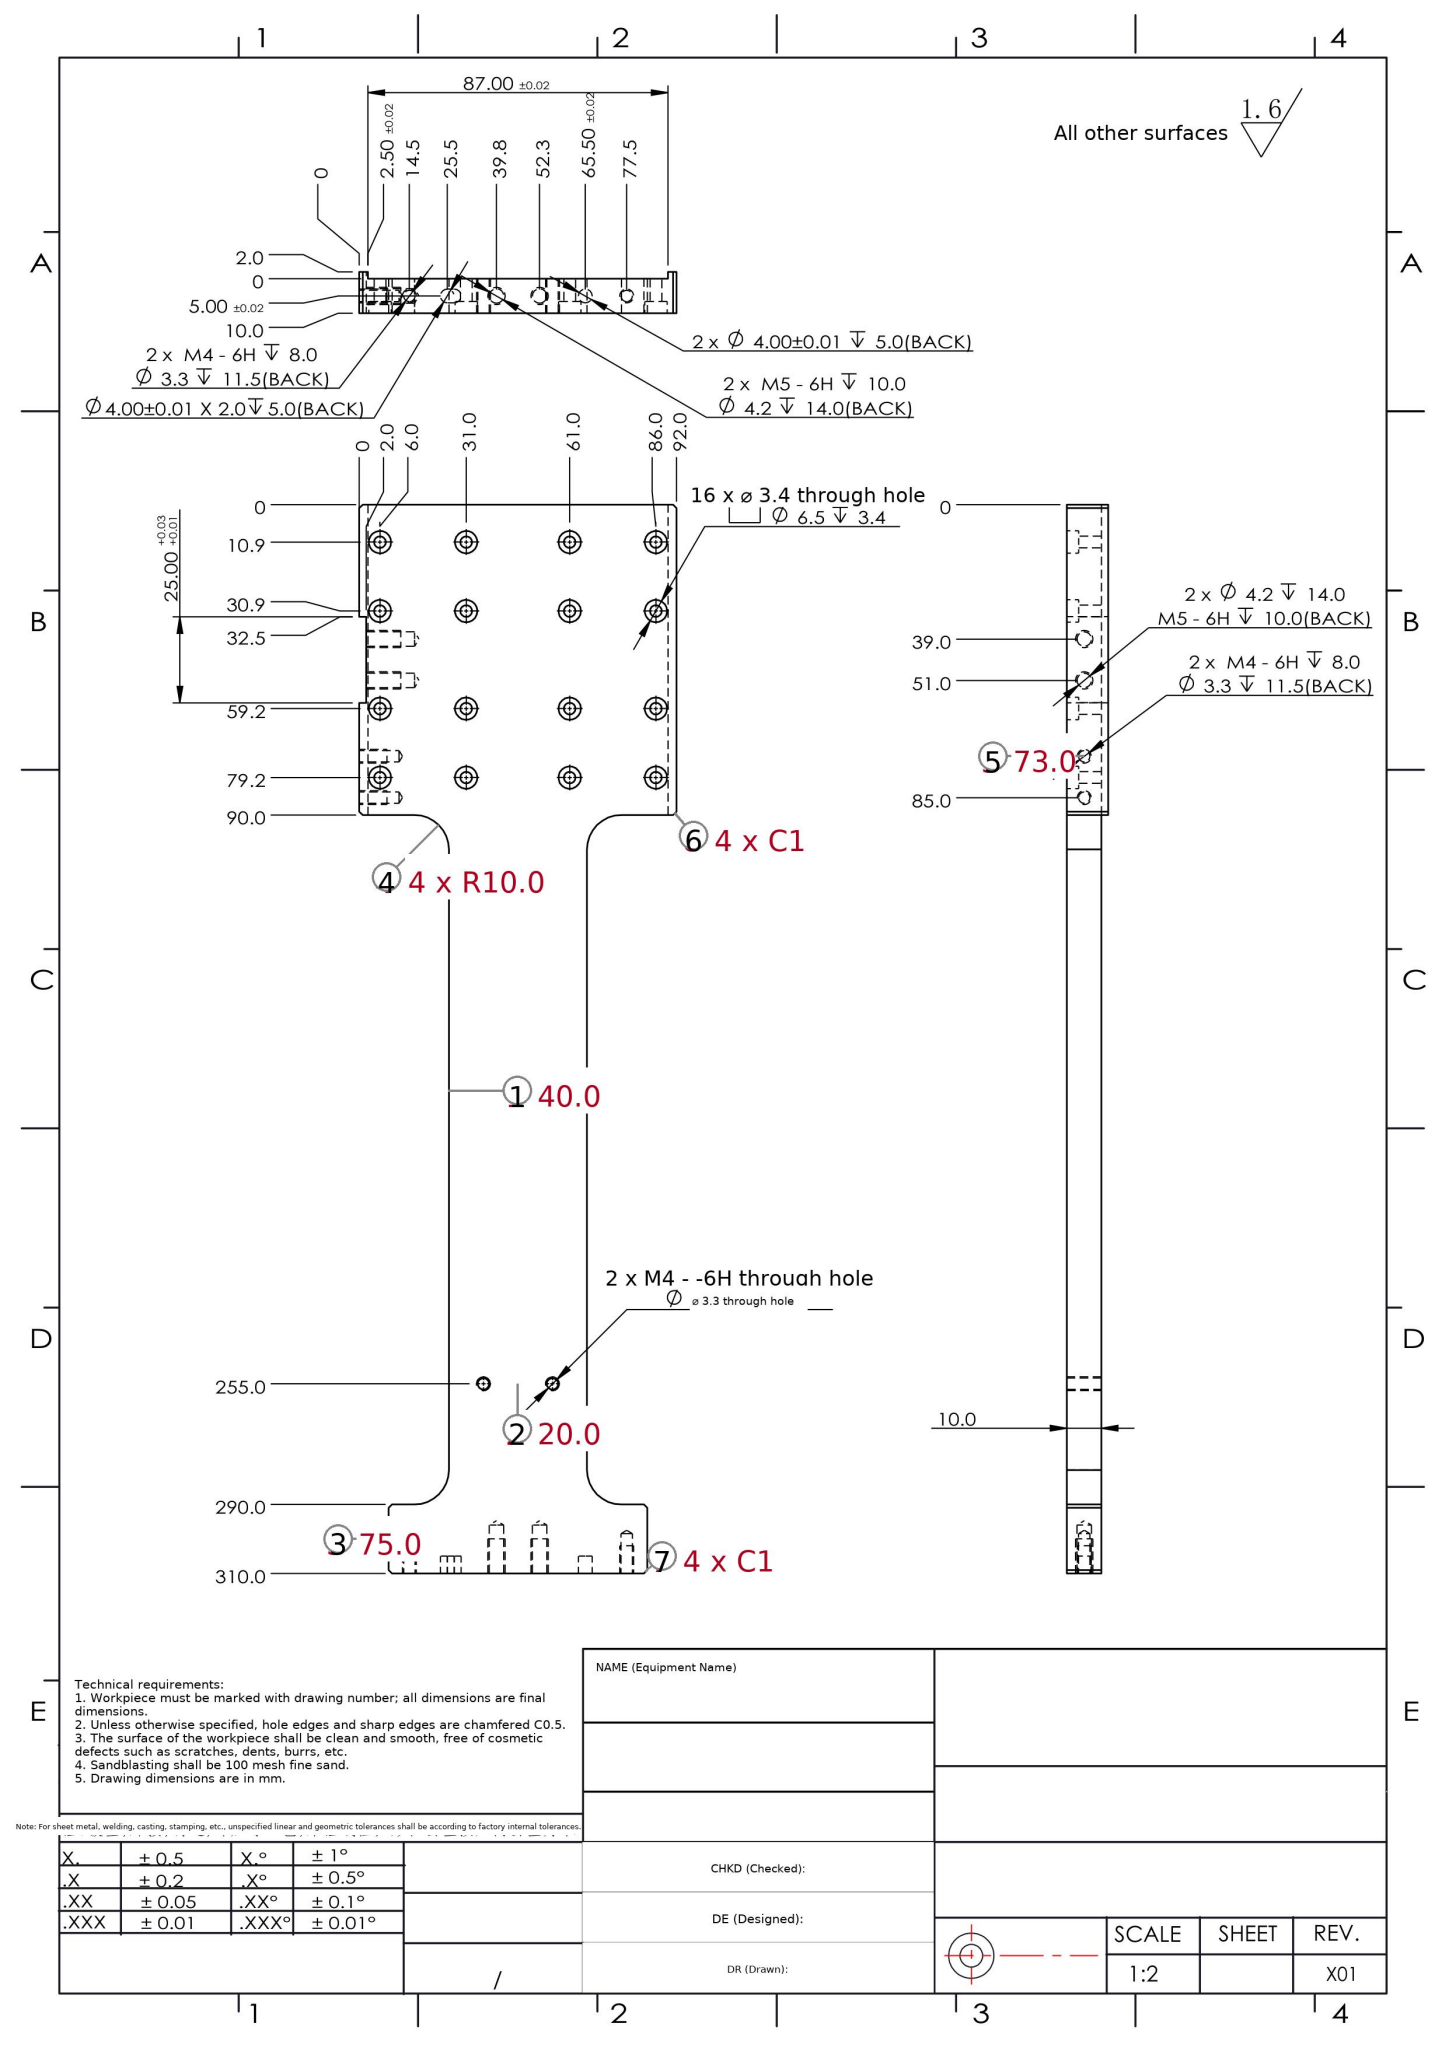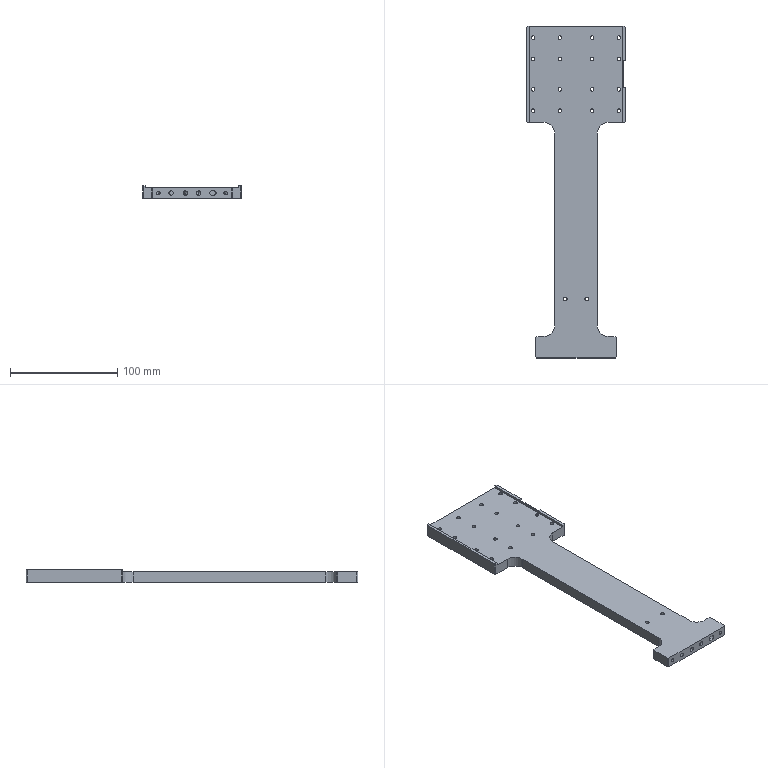Part | SolidWorks | mm | 1 solid | 158 faces | box 92 x 310 x 12 mm | volume 174610 mm3 | cylinder 92 | plane 50 | cone 16 | commonest cylinder face diameters 6.5 x32 3.4 x32 3.3 x12 4.2 x8 4 x4 20 x4